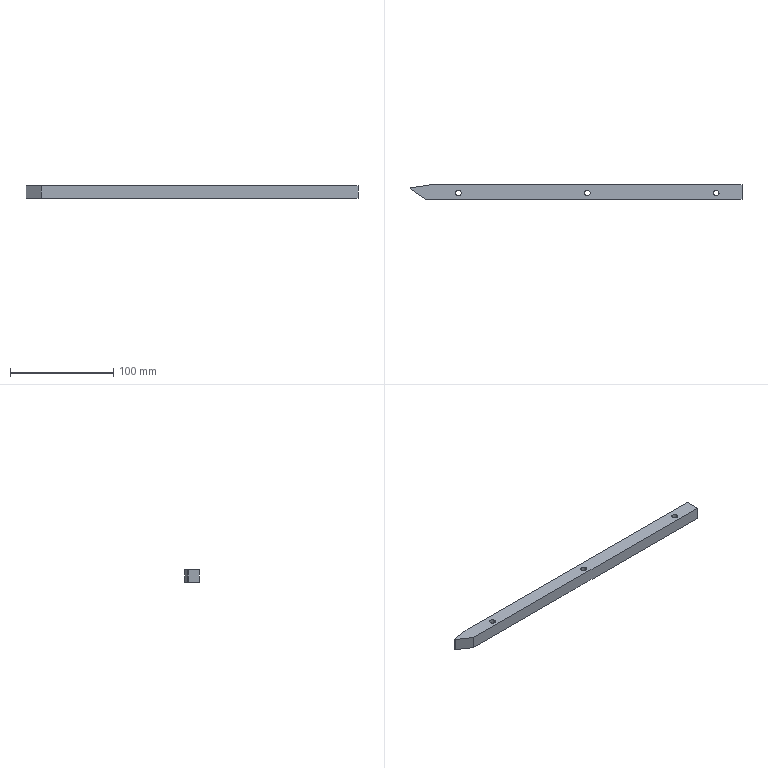Component | SolidWorks | OPW-05-014-1 | 1 solid | 23 faces | box 322 x 14 x 12 mm | volume 51159 mm3 | cylinder 12 | plane 11 | commonest cylinder face diameters 10 x6 5.5 x6
build123d program:
from build123d import *

# Parameters (mm, degrees)
SKETCH1_W                                       = 322
SKETCH1_H                                       = 14
BOSS_EXTRUDE1_DEPTH                             = 6
M5_HEX_SOCKET_HEAD_CAP_SCREW_CBORE1_D           = 5.5
M5_HEX_SOCKET_HEAD_CAP_SCREW_CBORE1_CBORE_D     = 10
M5_HEX_SOCKET_HEAD_CAP_SCREW_CBORE1_CBORE_DEPTH = 5
CHAMFER1_SIZE                                   = 3
CHAMFER1_SIZE2                                  = 20
CUT_EXTRUDE2_REACH                              = 163.598


with BuildPart() as part:
    # Sketch1 → Boss-Extrude1 (new, symmetric)
    with BuildSketch(Plane.XY):
        Rectangle(SKETCH1_W, SKETCH1_H)
    extrude(amount=BOSS_EXTRUDE1_DEPTH, both=True)

    # M5 Hex Socket Head Cap Screw CBORE1 (through all)
    with Locations(Plane.XY.offset(6)):
        with Locations((-136, -1), (-11, -1), (114, -1)):
            CounterBoreHole(M5_HEX_SOCKET_HEAD_CAP_SCREW_CBORE1_D / 2, M5_HEX_SOCKET_HEAD_CAP_SCREW_CBORE1_CBORE_D / 2, M5_HEX_SOCKET_HEAD_CAP_SCREW_CBORE1_CBORE_DEPTH)

    # Chamfer1
    chamfer1_edges = [part.edges().sort_by_distance(p)[0] for p in [
        (161, 7, 0),
    ]]
    chamfer1_side = [part.faces().sort_by_distance(p)[0] for p in [
        (161, 0, 0),
    ]]
    chamfer(chamfer1_edges, length=CHAMFER1_SIZE, length2=CHAMFER1_SIZE2, reference=chamfer1_side[0])

    # Sketch5 → Cut-Extrude2 (cut, up to next)
    with BuildSketch(Plane.XY.offset(6), mode=Mode.PRIVATE) as cut_extrude2_sk1:
        Polygon((161, 3), (146, -7), (161, -7), align=None)
    cut_extrude2_tool1 = extrude(cut_extrude2_sk1.sketch, amount=-CUT_EXTRUDE2_REACH, mode=Mode.PRIVATE) & part.part
    add(cut_extrude2_tool1.solids().sort_by_distance((156, -3.667, 6))[0], mode=Mode.SUBTRACT)


solid = part.part

# Placed as in the assembly
solid = solid.moved(Location((-115.904, 61.999, -46), (-180, 0, 180)))
STEP:
#1=CARTESIAN_POINT('',(0.988,2.402,-1.85));
#2=VERTEX_POINT('',#1);
#3=CARTESIAN_POINT('',(0.5943,2.402,-1.85));
#4=VERTEX_POINT('',#3);
#5=CARTESIAN_POINT('',(0.7912,2.402,-1.85));
#6=DIRECTION('',(-0.,-0.,-1.));
#7=DIRECTION('',(-1.,0.,0.));
#8=AXIS2_PLACEMENT_3D('',#5,#6,#7);
#9=CIRCLE('',#8,0.1969);
#10=EDGE_CURVE('',#2,#4,#9,.T.);
#11=ORIENTED_EDGE('',*,*,#10,.F.);
#12=CARTESIAN_POINT('',(0.988,2.402,-2.047));
#13=VERTEX_POINT('',#12);
#14=CARTESIAN_POINT('',(0.988,2.402,-2.047));
#15=DIRECTION('',(-0.,-0.,-1.));
#16=VECTOR('',#15,39.37);
#17=LINE('',#14,#16);
#18=EDGE_CURVE('',#2,#13,#17,.T.);
#19=ORIENTED_EDGE('',*,*,#18,.T.);
#20=CARTESIAN_POINT('',(0.5943,2.402,-2.047));
#21=VERTEX_POINT('',#20);
#22=CARTESIAN_POINT('',(0.7912,2.402,-2.047));
#23=DIRECTION('',(-0.,-0.,-1.));
#24=DIRECTION('',(-1.,0.,0.));
#25=AXIS2_PLACEMENT_3D('',#22,#23,#24);
#26=CIRCLE('',#25,0.1969);
#27=EDGE_CURVE('',#13,#21,#26,.T.);
#28=ORIENTED_EDGE('',*,*,#27,.T.);
#29=CARTESIAN_POINT('',(0.5943,2.402,-2.047));
#30=DIRECTION('',(-0.,-0.,-1.));
#31=VECTOR('',#30,39.37);
#32=LINE('',#29,#31);
#33=EDGE_CURVE('',#4,#21,#32,.T.);
#34=ORIENTED_EDGE('',*,*,#33,.F.);
#35=EDGE_LOOP('',(#11,#19,#28,#34));
#36=FACE_OUTER_BOUND('',#35,.T.);
#37=CARTESIAN_POINT('',(0.7912,2.402,-2.047));
#38=DIRECTION('',(-0.,-0.,-1.));
#39=DIRECTION('',(-1.,0.,0.));
#40=AXIS2_PLACEMENT_3D('',#37,#38,#39);
#41=CYLINDRICAL_SURFACE('',#40,0.1969);
#42=ADVANCED_FACE('',(#36),#41,.F.);
#43=CARTESIAN_POINT('',(0.8995,2.402,-1.575));
#44=VERTEX_POINT('',#43);
#45=CARTESIAN_POINT('',(0.6829,2.402,-1.575));
#46=VERTEX_POINT('',#45);
#47=CARTESIAN_POINT('',(0.7912,2.402,-1.575));
#48=DIRECTION('',(-0.,-0.,-1.));
#49=DIRECTION('',(-1.,0.,0.));
#50=AXIS2_PLACEMENT_3D('',#47,#48,#49);
#51=CIRCLE('',#50,0.1083);
#52=EDGE_CURVE('',#44,#46,#51,.T.);
#53=ORIENTED_EDGE('',*,*,#52,.F.);
#54=CARTESIAN_POINT('',(0.8995,2.402,-1.85));
#55=VERTEX_POINT('',#54);
#56=CARTESIAN_POINT('',(0.8995,2.402,-2.047));
#57=DIRECTION('',(-0.,-0.,-1.));
#58=VECTOR('',#57,39.37);
#59=LINE('',#56,#58);
#60=EDGE_CURVE('',#44,#55,#59,.T.);
#61=ORIENTED_EDGE('',*,*,#60,.T.);
#62=CARTESIAN_POINT('',(0.6829,2.402,-1.85));
#63=VERTEX_POINT('',#62);
#64=CARTESIAN_POINT('',(0.7912,2.402,-1.85));
#65=DIRECTION('',(-0.,-0.,-1.));
#66=DIRECTION('',(-1.,0.,0.));
#67=AXIS2_PLACEMENT_3D('',#64,#65,#66);
#68=CIRCLE('',#67,0.1083);
#69=EDGE_CURVE('',#55,#63,#68,.T.);
#70=ORIENTED_EDGE('',*,*,#69,.T.);
#71=CARTESIAN_POINT('',(0.6829,2.402,-2.047));
#72=DIRECTION('',(-0.,-0.,-1.));
#73=VECTOR('',#72,39.37);
#74=LINE('',#71,#73);
#75=EDGE_CURVE('',#46,#63,#74,.T.);
#76=ORIENTED_EDGE('',*,*,#75,.F.);
#77=EDGE_LOOP('',(#53,#61,#70,#76));
#78=FACE_OUTER_BOUND('',#77,.T.);
#79=CARTESIAN_POINT('',(0.7912,2.402,-2.047));
#80=DIRECTION('',(-0.,-0.,-1.));
#81=DIRECTION('',(-1.,0.,0.));
#82=AXIS2_PLACEMENT_3D('',#79,#80,#81);
#83=CYLINDRICAL_SURFACE('',#82,0.1083);
#84=ADVANCED_FACE('',(#78),#83,.F.);
#85=CARTESIAN_POINT('',(-3.933,2.402,-1.85));
#86=VERTEX_POINT('',#85);
#87=CARTESIAN_POINT('',(-4.327,2.402,-1.85));
#88=VERTEX_POINT('',#87);
#89=CARTESIAN_POINT('',(-4.13,2.402,-1.85));
#90=DIRECTION('',(-0.,-0.,-1.));
#91=DIRECTION('',(-1.,0.,0.));
#92=AXIS2_PLACEMENT_3D('',#89,#90,#91);
#93=CIRCLE('',#92,0.1969);
#94=EDGE_CURVE('',#86,#88,#93,.T.);
#95=ORIENTED_EDGE('',*,*,#94,.F.);
#96=CARTESIAN_POINT('',(-3.933,2.402,-2.047));
#97=VERTEX_POINT('',#96);
#98=CARTESIAN_POINT('',(-3.933,2.402,-2.047));
#99=DIRECTION('',(-0.,-0.,-1.));
#100=VECTOR('',#99,39.37);
#101=LINE('',#98,#100);
#102=EDGE_CURVE('',#86,#97,#101,.T.);
#103=ORIENTED_EDGE('',*,*,#102,.T.);
#104=CARTESIAN_POINT('',(-4.327,2.402,-2.047));
#105=VERTEX_POINT('',#104);
#106=CARTESIAN_POINT('',(-4.13,2.402,-2.047));
#107=DIRECTION('',(-0.,-0.,-1.));
#108=DIRECTION('',(-1.,0.,0.));
#109=AXIS2_PLACEMENT_3D('',#106,#107,#108);
#110=CIRCLE('',#109,0.1969);
#111=EDGE_CURVE('',#97,#105,#110,.T.);
#112=ORIENTED_EDGE('',*,*,#111,.T.);
#113=CARTESIAN_POINT('',(-4.327,2.402,-2.047));
#114=DIRECTION('',(-0.,-0.,-1.));
#115=VECTOR('',#114,39.37);
#116=LINE('',#113,#115);
#117=EDGE_CURVE('',#88,#105,#116,.T.);
#118=ORIENTED_EDGE('',*,*,#117,.F.);
#119=EDGE_LOOP('',(#95,#103,#112,#118));
#120=FACE_OUTER_BOUND('',#119,.T.);
#121=CARTESIAN_POINT('',(-4.13,2.402,-2.047));
#122=DIRECTION('',(-0.,-0.,-1.));
#123=DIRECTION('',(-1.,0.,0.));
#124=AXIS2_PLACEMENT_3D('',#121,#122,#123);
#125=CYLINDRICAL_SURFACE('',#124,0.1969);
#126=ADVANCED_FACE('',(#120),#125,.F.);
#127=CARTESIAN_POINT('',(-4.022,2.402,-1.575));
#128=VERTEX_POINT('',#127);
#129=CARTESIAN_POINT('',(-4.238,2.402,-1.575));
#130=VERTEX_POINT('',#129);
#131=CARTESIAN_POINT('',(-4.13,2.402,-1.575));
#132=DIRECTION('',(-0.,-0.,-1.));
#133=DIRECTION('',(-1.,0.,0.));
#134=AXIS2_PLACEMENT_3D('',#131,#132,#133);
#135=CIRCLE('',#134,0.1083);
#136=EDGE_CURVE('',#128,#130,#135,.T.);
#137=ORIENTED_EDGE('',*,*,#136,.F.);
#138=CARTESIAN_POINT('',(-4.022,2.402,-1.85));
#139=VERTEX_POINT('',#138);
#140=CARTESIAN_POINT('',(-4.022,2.402,-2.047));
#141=DIRECTION('',(-0.,-0.,-1.));
#142=VECTOR('',#141,39.37);
#143=LINE('',#140,#142);
#144=EDGE_CURVE('',#128,#139,#143,.T.);
#145=ORIENTED_EDGE('',*,*,#144,.T.);
#146=CARTESIAN_POINT('',(-4.238,2.402,-1.85));
#147=VERTEX_POINT('',#146);
#148=CARTESIAN_POINT('',(-4.13,2.402,-1.85));
#149=DIRECTION('',(-0.,-0.,-1.));
#150=DIRECTION('',(-1.,0.,0.));
#151=AXIS2_PLACEMENT_3D('',#148,#149,#150);
#152=CIRCLE('',#151,0.1083);
#153=EDGE_CURVE('',#139,#147,#152,.T.);
#154=ORIENTED_EDGE('',*,*,#153,.T.);
#155=CARTESIAN_POINT('',(-4.238,2.402,-2.047));
#156=DIRECTION('',(-0.,-0.,-1.));
#157=VECTOR('',#156,39.37);
#158=LINE('',#155,#157);
#159=EDGE_CURVE('',#130,#147,#158,.T.);
#160=ORIENTED_EDGE('',*,*,#159,.F.);
#161=EDGE_LOOP('',(#137,#145,#154,#160));
#162=FACE_OUTER_BOUND('',#161,.T.);
#163=CARTESIAN_POINT('',(-4.13,2.402,-2.047));
#164=DIRECTION('',(-0.,-0.,-1.));
#165=DIRECTION('',(-1.,0.,0.));
#166=AXIS2_PLACEMENT_3D('',#163,#164,#165);
#167=CYLINDRICAL_SURFACE('',#166,0.1083);
#168=ADVANCED_FACE('',(#162),#167,.F.);
#169=CARTESIAN_POINT('',(-8.854,2.402,-1.85));
#170=VERTEX_POINT('',#169);
#171=CARTESIAN_POINT('',(-9.248,2.402,-1.85));
#172=VERTEX_POINT('',#171);
#173=CARTESIAN_POINT('',(-9.051,2.402,-1.85));
#174=DIRECTION('',(-0.,-0.,-1.));
#175=DIRECTION('',(-1.,0.,0.));
#176=AXIS2_PLACEMENT_3D('',#173,#174,#175);
#177=CIRCLE('',#176,0.1969);
#178=EDGE_CURVE('',#170,#172,#177,.T.);
#179=ORIENTED_EDGE('',*,*,#178,.F.);
#180=CARTESIAN_POINT('',(-8.854,2.402,-2.047));
#181=VERTEX_POINT('',#180);
#182=CARTESIAN_POINT('',(-8.854,2.402,-2.047));
#183=DIRECTION('',(-0.,-0.,-1.));
#184=VECTOR('',#183,39.37);
#185=LINE('',#182,#184);
#186=EDGE_CURVE('',#170,#181,#185,.T.);
#187=ORIENTED_EDGE('',*,*,#186,.T.);
#188=CARTESIAN_POINT('',(-9.248,2.402,-2.047));
#189=VERTEX_POINT('',#188);
#190=CARTESIAN_POINT('',(-9.051,2.402,-2.047));
#191=DIRECTION('',(-0.,-0.,-1.));
#192=DIRECTION('',(-1.,0.,0.));
#193=AXIS2_PLACEMENT_3D('',#190,#191,#192);
#194=CIRCLE('',#193,0.1969);
#195=EDGE_CURVE('',#181,#189,#194,.T.);
#196=ORIENTED_EDGE('',*,*,#195,.T.);
#197=CARTESIAN_POINT('',(-9.248,2.402,-2.047));
#198=DIRECTION('',(-0.,-0.,-1.));
#199=VECTOR('',#198,39.37);
#200=LINE('',#197,#199);
#201=EDGE_CURVE('',#172,#189,#200,.T.);
#202=ORIENTED_EDGE('',*,*,#201,.F.);
#203=EDGE_LOOP('',(#179,#187,#196,#202));
#204=FACE_OUTER_BOUND('',#203,.T.);
#205=CARTESIAN_POINT('',(-9.051,2.402,-2.047));
#206=DIRECTION('',(-0.,-0.,-1.));
#207=DIRECTION('',(-1.,0.,0.));
#208=AXIS2_PLACEMENT_3D('',#205,#206,#207);
#209=CYLINDRICAL_SURFACE('',#208,0.1969);
#210=ADVANCED_FACE('',(#204),#209,.F.);
#211=CARTESIAN_POINT('',(-8.943,2.402,-1.575));
#212=VERTEX_POINT('',#211);
#213=CARTESIAN_POINT('',(-9.16,2.402,-1.575));
#214=VERTEX_POINT('',#213);
#215=CARTESIAN_POINT('',(-9.051,2.402,-1.575));
#216=DIRECTION('',(-0.,-0.,-1.));
#217=DIRECTION('',(-1.,0.,0.));
#218=AXIS2_PLACEMENT_3D('',#215,#216,#217);
#219=CIRCLE('',#218,0.1083);
#220=EDGE_CURVE('',#212,#214,#219,.T.);
#221=ORIENTED_EDGE('',*,*,#220,.F.);
#222=CARTESIAN_POINT('',(-8.943,2.402,-1.85));
#223=VERTEX_POINT('',#222);
#224=CARTESIAN_POINT('',(-8.943,2.402,-2.047));
#225=DIRECTION('',(-0.,-0.,-1.));
#226=VECTOR('',#225,39.37);
#227=LINE('',#224,#226);
#228=EDGE_CURVE('',#212,#223,#227,.T.);
#229=ORIENTED_EDGE('',*,*,#228,.T.);
#230=CARTESIAN_POINT('',(-9.16,2.402,-1.85));
#231=VERTEX_POINT('',#230);
#232=CARTESIAN_POINT('',(-9.051,2.402,-1.85));
#233=DIRECTION('',(-0.,-0.,-1.));
#234=DIRECTION('',(-1.,0.,0.));
#235=AXIS2_PLACEMENT_3D('',#232,#233,#234);
#236=CIRCLE('',#235,0.1083);
#237=EDGE_CURVE('',#223,#231,#236,.T.);
#238=ORIENTED_EDGE('',*,*,#237,.T.);
#239=CARTESIAN_POINT('',(-9.16,2.402,-2.047));
#240=DIRECTION('',(-0.,-0.,-1.));
#241=VECTOR('',#240,39.37);
#242=LINE('',#239,#241);
#243=EDGE_CURVE('',#214,#231,#242,.T.);
#244=ORIENTED_EDGE('',*,*,#243,.F.);
#245=EDGE_LOOP('',(#221,#229,#238,#244));
#246=FACE_OUTER_BOUND('',#245,.T.);
#247=CARTESIAN_POINT('',(-9.051,2.402,-2.047));
#248=DIRECTION('',(-0.,-0.,-1.));
#249=DIRECTION('',(-1.,0.,0.));
#250=AXIS2_PLACEMENT_3D('',#247,#248,#249);
#251=CYLINDRICAL_SURFACE('',#250,0.1083);
#252=ADVANCED_FACE('',(#246),#251,.F.);
#253=CARTESIAN_POINT('',(1.775,2.716,-1.575));
#254=VERTEX_POINT('',#253);
#255=CARTESIAN_POINT('',(1.775,2.165,-1.575));
#256=VERTEX_POINT('',#255);
#257=CARTESIAN_POINT('',(1.775,2.716,-1.575));
#258=DIRECTION('',(-0.,-1.,0.));
#259=VECTOR('',#258,39.37);
#260=LINE('',#257,#259);
#261=EDGE_CURVE('',#254,#256,#260,.T.);
#262=ORIENTED_EDGE('',*,*,#261,.T.);
#263=CARTESIAN_POINT('',(1.775,2.165,-2.047));
#264=VERTEX_POINT('',#263);
#265=CARTESIAN_POINT('',(1.775,2.165,-2.047));
#266=DIRECTION('',(0.,0.,1.));
#267=VECTOR('',#266,39.37);
#268=LINE('',#265,#267);
#269=EDGE_CURVE('',#264,#256,#268,.T.);
#270=ORIENTED_EDGE('',*,*,#269,.F.);
#271=CARTESIAN_POINT('',(1.775,2.716,-2.047));
#272=VERTEX_POINT('',#271);
#273=CARTESIAN_POINT('',(1.775,2.716,-2.047));
#274=DIRECTION('',(-0.,-1.,0.));
#275=VECTOR('',#274,39.37);
#276=LINE('',#273,#275);
#277=EDGE_CURVE('',#272,#264,#276,.T.);
#278=ORIENTED_EDGE('',*,*,#277,.F.);
#279=CARTESIAN_POINT('',(1.775,2.716,-2.047));
#280=DIRECTION('',(0.,0.,1.));
#281=VECTOR('',#280,39.37);
#282=LINE('',#279,#281);
#283=EDGE_CURVE('',#272,#254,#282,.T.);
#284=ORIENTED_EDGE('',*,*,#283,.T.);
#285=EDGE_LOOP('',(#262,#270,#278,#284));
#286=FACE_OUTER_BOUND('',#285,.T.);
#287=CARTESIAN_POINT('',(1.775,2.716,-2.047));
#288=DIRECTION('',(-1.,0.,0.));
#289=DIRECTION('',(0.,0.,1.));
#290=AXIS2_PLACEMENT_3D('',#287,#288,#289);
#291=PLANE('',#290);
#292=ADVANCED_FACE('',(#286),#291,.F.);
#293=CARTESIAN_POINT('',(-10.311,2.165,-1.575));
#294=VERTEX_POINT('',#293);
#295=CARTESIAN_POINT('',(1.775,2.165,-1.575));
#296=DIRECTION('',(-1.,0.,-0.));
#297=VECTOR('',#296,39.37);
#298=LINE('',#295,#297);
#299=EDGE_CURVE('',#256,#294,#298,.T.);
#300=ORIENTED_EDGE('',*,*,#299,.T.);
#301=CARTESIAN_POINT('',(-10.311,2.165,-2.047));
#302=VERTEX_POINT('',#301);
#303=CARTESIAN_POINT('',(-10.311,2.165,-1.575));
#304=DIRECTION('',(-0.,-0.,-1.));
#305=VECTOR('',#304,39.37);
#306=LINE('',#303,#305);
#307=EDGE_CURVE('',#294,#302,#306,.T.);
#308=ORIENTED_EDGE('',*,*,#307,.T.);
#309=CARTESIAN_POINT('',(1.775,2.165,-2.047));
#310=DIRECTION('',(-1.,0.,-0.));
#311=VECTOR('',#310,39.37);
#312=LINE('',#309,#311);
#313=EDGE_CURVE('',#264,#302,#312,.T.);
#314=ORIENTED_EDGE('',*,*,#313,.F.);
#315=ORIENTED_EDGE('',*,*,#269,.T.);
#316=EDGE_LOOP('',(#300,#308,#314,#315));
#317=FACE_OUTER_BOUND('',#316,.T.);
#318=CARTESIAN_POINT('',(1.775,2.165,-2.047));
#319=DIRECTION('',(0.,1.,-0.));
#320=DIRECTION('',(1.,-0.,0.));
#321=AXIS2_PLACEMENT_3D('',#318,#319,#320);
#322=PLANE('',#321);
#323=ADVANCED_FACE('',(#317),#322,.F.);
#324=CARTESIAN_POINT('',(-10.902,2.559,-2.047));
#325=VERTEX_POINT('',#324);
#326=CARTESIAN_POINT('',(-10.902,2.598,-2.047));
#327=VERTEX_POINT('',#326);
#328=CARTESIAN_POINT('',(-10.902,2.716,-2.047));
#329=DIRECTION('',(0.,1.,-0.));
#330=VECTOR('',#329,39.37);
#331=LINE('',#328,#330);
#332=EDGE_CURVE('',#325,#327,#331,.T.);
#333=ORIENTED_EDGE('',*,*,#332,.F.);
#334=CARTESIAN_POINT('',(-10.902,2.559,-1.575));
#335=VERTEX_POINT('',#334);
#336=CARTESIAN_POINT('',(-10.902,2.559,-1.575));
#337=DIRECTION('',(-0.,-0.,-1.));
#338=VECTOR('',#337,39.37);
#339=LINE('',#336,#338);
#340=EDGE_CURVE('',#335,#325,#339,.T.);
#341=ORIENTED_EDGE('',*,*,#340,.F.);
#342=CARTESIAN_POINT('',(-10.902,2.598,-1.575));
#343=VERTEX_POINT('',#342);
#344=CARTESIAN_POINT('',(-10.902,2.716,-1.575));
#345=DIRECTION('',(0.,1.,-0.));
#346=VECTOR('',#345,39.37);
#347=LINE('',#344,#346);
#348=EDGE_CURVE('',#335,#343,#347,.T.);
#349=ORIENTED_EDGE('',*,*,#348,.T.);
#350=CARTESIAN_POINT('',(-10.902,2.598,-2.047));
#351=DIRECTION('',(-0.,-0.,-1.));
#352=VECTOR('',#351,39.37);
#353=LINE('',#350,#352);
#354=EDGE_CURVE('',#343,#327,#353,.T.);
#355=ORIENTED_EDGE('',*,*,#354,.T.);
#356=EDGE_LOOP('',(#333,#341,#349,#355));
#357=FACE_OUTER_BOUND('',#356,.T.);
#358=CARTESIAN_POINT('',(-10.902,2.716,-2.047));
#359=DIRECTION('',(1.,-0.,-0.));
#360=DIRECTION('',(-0.,-0.,-1.));
#361=AXIS2_PLACEMENT_3D('',#358,#359,#360);
#362=PLANE('',#361);
#363=ADVANCED_FACE('',(#357),#362,.F.);
#364=CARTESIAN_POINT('',(-10.114,2.716,-2.047));
#365=VERTEX_POINT('',#364);
#366=CARTESIAN_POINT('',(1.775,2.716,-2.047));
#367=DIRECTION('',(1.,-0.,0.));
#368=VECTOR('',#367,39.37);
#369=LINE('',#366,#368);
#370=EDGE_CURVE('',#365,#272,#369,.T.);
#371=ORIENTED_EDGE('',*,*,#370,.F.);
#372=CARTESIAN_POINT('',(-10.114,2.716,-1.575));
#373=VERTEX_POINT('',#372);
#374=CARTESIAN_POINT('',(-10.114,2.716,-2.047));
#375=DIRECTION('',(0.,0.,1.));
#376=VECTOR('',#375,39.37);
#377=LINE('',#374,#376);
#378=EDGE_CURVE('',#365,#373,#377,.T.);
#379=ORIENTED_EDGE('',*,*,#378,.T.);
#380=CARTESIAN_POINT('',(1.775,2.716,-1.575));
#381=DIRECTION('',(1.,-0.,0.));
#382=VECTOR('',#381,39.37);
#383=LINE('',#380,#382);
#384=EDGE_CURVE('',#373,#254,#383,.T.);
#385=ORIENTED_EDGE('',*,*,#384,.T.);
#386=ORIENTED_EDGE('',*,*,#283,.F.);
#387=EDGE_LOOP('',(#371,#379,#385,#386));
#388=FACE_OUTER_BOUND('',#387,.T.);
#389=CARTESIAN_POINT('',(1.775,2.716,-2.047));
#390=DIRECTION('',(-0.,-1.,0.));
#391=DIRECTION('',(-1.,0.,-0.));
#392=AXIS2_PLACEMENT_3D('',#389,#390,#391);
#393=PLANE('',#392);
#394=ADVANCED_FACE('',(#388),#393,.F.);
#395=CARTESIAN_POINT('',(-10.902,2.559,-2.047));
#396=DIRECTION('',(0.8321,-0.5547,0.));
#397=VECTOR('',#396,39.37);
#398=LINE('',#395,#397);
#399=EDGE_CURVE('',#325,#302,#398,.T.);
#400=ORIENTED_EDGE('',*,*,#399,.F.);
#401=ORIENTED_EDGE('',*,*,#332,.T.);
#402=CARTESIAN_POINT('',(1.433,4.449,-2.047));
#403=DIRECTION('',(0.9889,0.1483,0.));
#404=VECTOR('',#403,39.37);
#405=LINE('',#402,#404);
#406=EDGE_CURVE('',#327,#365,#405,.T.);
#407=ORIENTED_EDGE('',*,*,#406,.T.);
#408=ORIENTED_EDGE('',*,*,#370,.T.);
#409=ORIENTED_EDGE('',*,*,#277,.T.);
#410=ORIENTED_EDGE('',*,*,#313,.T.);
#411=EDGE_LOOP('',(#400,#401,#407,#408,#409,#410));
#412=FACE_OUTER_BOUND('',#411,.T.);
#413=CARTESIAN_POINT('',(0.7912,2.402,-2.047));
#414=DIRECTION('',(-0.,-0.,-1.));
#415=DIRECTION('',(-1.,0.,0.));
#416=AXIS2_PLACEMENT_3D('',#413,#414,#415);
#417=CIRCLE('',#416,0.1969);
#418=EDGE_CURVE('',#21,#13,#417,.T.);
#419=ORIENTED_EDGE('',*,*,#418,.F.);
#420=ORIENTED_EDGE('',*,*,#27,.F.);
#421=EDGE_LOOP('',(#419,#420));
#422=FACE_BOUND('',#421,.T.);
#423=CARTESIAN_POINT('',(-4.13,2.402,-2.047));
#424=DIRECTION('',(-0.,-0.,-1.));
#425=DIRECTION('',(-1.,0.,0.));
#426=AXIS2_PLACEMENT_3D('',#423,#424,#425);
#427=CIRCLE('',#426,0.1969);
#428=EDGE_CURVE('',#105,#97,#427,.T.);
#429=ORIENTED_EDGE('',*,*,#428,.F.);
#430=ORIENTED_EDGE('',*,*,#111,.F.);
#431=EDGE_LOOP('',(#429,#430));
#432=FACE_BOUND('',#431,.T.);
#433=CARTESIAN_POINT('',(-9.051,2.402,-2.047));
#434=DIRECTION('',(-0.,-0.,-1.));
#435=DIRECTION('',(-1.,0.,0.));
#436=AXIS2_PLACEMENT_3D('',#433,#434,#435);
#437=CIRCLE('',#436,0.1969);
#438=EDGE_CURVE('',#189,#181,#437,.T.);
#439=ORIENTED_EDGE('',*,*,#438,.F.);
#440=ORIENTED_EDGE('',*,*,#195,.F.);
#441=EDGE_LOOP('',(#439,#440));
#442=FACE_BOUND('',#441,.T.);
#443=CARTESIAN_POINT('',(1.775,2.165,-2.047));
#444=DIRECTION('',(0.,-0.,-1.));
#445=DIRECTION('',(-1.,0.,-0.));
#446=AXIS2_PLACEMENT_3D('',#443,#444,#445);
#447=PLANE('',#446);
#448=ADVANCED_FACE('',(#412,#422,#432,#442),#447,.T.);
#449=CARTESIAN_POINT('',(0.7912,2.402,-1.575));
#450=DIRECTION('',(-0.,-0.,-1.));
#451=DIRECTION('',(-1.,0.,0.));
#452=AXIS2_PLACEMENT_3D('',#449,#450,#451);
#453=CIRCLE('',#452,0.1083);
#454=EDGE_CURVE('',#46,#44,#453,.T.);
#455=ORIENTED_EDGE('',*,*,#454,.T.);
#456=ORIENTED_EDGE('',*,*,#52,.T.);
#457=EDGE_LOOP('',(#455,#456));
#458=FACE_BOUND('',#457,.T.);
#459=CARTESIAN_POINT('',(-4.13,2.402,-1.575));
#460=DIRECTION('',(-0.,-0.,-1.));
#461=DIRECTION('',(-1.,0.,0.));
#462=AXIS2_PLACEMENT_3D('',#459,#460,#461);
#463=CIRCLE('',#462,0.1083);
#464=EDGE_CURVE('',#130,#128,#463,.T.);
#465=ORIENTED_EDGE('',*,*,#464,.T.);
#466=ORIENTED_EDGE('',*,*,#136,.T.);
#467=EDGE_LOOP('',(#465,#466));
#468=FACE_BOUND('',#467,.T.);
#469=CARTESIAN_POINT('',(-9.051,2.402,-1.575));
#470=DIRECTION('',(-0.,-0.,-1.));
#471=DIRECTION('',(-1.,0.,0.));
#472=AXIS2_PLACEMENT_3D('',#469,#470,#471);
#473=CIRCLE('',#472,0.1083);
#474=EDGE_CURVE('',#214,#212,#473,.T.);
#475=ORIENTED_EDGE('',*,*,#474,.T.);
#476=ORIENTED_EDGE('',*,*,#220,.T.);
#477=EDGE_LOOP('',(#475,#476));
#478=FACE_BOUND('',#477,.T.);
#479=ORIENTED_EDGE('',*,*,#348,.F.);
#480=CARTESIAN_POINT('',(-10.902,2.559,-1.575));
#481=DIRECTION('',(-0.8321,0.5547,-0.));
#482=VECTOR('',#481,39.37);
#483=LINE('',#480,#482);
#484=EDGE_CURVE('',#294,#335,#483,.T.);
#485=ORIENTED_EDGE('',*,*,#484,.F.);
#486=ORIENTED_EDGE('',*,*,#299,.F.);
#487=ORIENTED_EDGE('',*,*,#261,.F.);
#488=ORIENTED_EDGE('',*,*,#384,.F.);
#489=CARTESIAN_POINT('',(-10.114,2.716,-1.575));
#490=DIRECTION('',(-0.9889,-0.1483,-0.));
#491=VECTOR('',#490,39.37);
#492=LINE('',#489,#491);
#493=EDGE_CURVE('',#373,#343,#492,.T.);
#494=ORIENTED_EDGE('',*,*,#493,.T.);
#495=EDGE_LOOP('',(#479,#485,#486,#487,#488,#494));
#496=FACE_OUTER_BOUND('',#495,.T.);
#497=CARTESIAN_POINT('',(1.775,2.165,-1.575));
#498=DIRECTION('',(0.,-0.,-1.));
#499=DIRECTION('',(-1.,0.,-0.));
#500=AXIS2_PLACEMENT_3D('',#497,#498,#499);
#501=PLANE('',#500);
#502=ADVANCED_FACE('',(#458,#468,#478,#496),#501,.F.);
#503=ORIENTED_EDGE('',*,*,#228,.F.);
#504=ORIENTED_EDGE('',*,*,#474,.F.);
#505=ORIENTED_EDGE('',*,*,#243,.T.);
#506=CARTESIAN_POINT('',(-9.051,2.402,-1.85));
#507=DIRECTION('',(-0.,-0.,-1.));
#508=DIRECTION('',(-1.,0.,0.));
#509=AXIS2_PLACEMENT_3D('',#506,#507,#508);
#510=CIRCLE('',#509,0.1083);
#511=EDGE_CURVE('',#231,#223,#510,.T.);
#512=ORIENTED_EDGE('',*,*,#511,.T.);
#513=EDGE_LOOP('',(#503,#504,#505,#512));
#514=FACE_OUTER_BOUND('',#513,.T.);
#515=CARTESIAN_POINT('',(-9.051,2.402,-2.047));
#516=DIRECTION('',(-0.,-0.,-1.));
#517=DIRECTION('',(-1.,0.,0.));
#518=AXIS2_PLACEMENT_3D('',#515,#516,#517);
#519=CYLINDRICAL_SURFACE('',#518,0.1083);
#520=ADVANCED_FACE('',(#514),#519,.F.);
#521=ORIENTED_EDGE('',*,*,#511,.F.);
#522=ORIENTED_EDGE('',*,*,#237,.F.);
#523=EDGE_LOOP('',(#521,#522));
#524=FACE_BOUND('',#523,.T.);
#525=CARTESIAN_POINT('',(-9.051,2.402,-1.85));
#526=DIRECTION('',(-0.,-0.,-1.));
#527=DIRECTION('',(-1.,0.,0.));
#528=AXIS2_PLACEMENT_3D('',#525,#526,#527);
#529=CIRCLE('',#528,0.1969);
#530=EDGE_CURVE('',#172,#170,#529,.T.);
#531=ORIENTED_EDGE('',*,*,#530,.T.);
#532=ORIENTED_EDGE('',*,*,#178,.T.);
#533=EDGE_LOOP('',(#531,#532));
#534=FACE_OUTER_BOUND('',#533,.T.);
#535=CARTESIAN_POINT('',(-9.16,2.402,-1.85));
#536=DIRECTION('',(-0.,0.,1.));
#537=DIRECTION('',(1.,-0.,0.));
#538=AXIS2_PLACEMENT_3D('',#535,#536,#537);
#539=PLANE('',#538);
#540=ADVANCED_FACE('',(#524,#534),#539,.F.);
#541=ORIENTED_EDGE('',*,*,#186,.F.);
#542=ORIENTED_EDGE('',*,*,#530,.F.);
#543=ORIENTED_EDGE('',*,*,#201,.T.);
#544=ORIENTED_EDGE('',*,*,#438,.T.);
#545=EDGE_LOOP('',(#541,#542,#543,#544));
#546=FACE_OUTER_BOUND('',#545,.T.);
#547=CARTESIAN_POINT('',(-9.051,2.402,-2.047));
#548=DIRECTION('',(-0.,-0.,-1.));
#549=DIRECTION('',(-1.,0.,0.));
#550=AXIS2_PLACEMENT_3D('',#547,#548,#549);
#551=CYLINDRICAL_SURFACE('',#550,0.1969);
#552=ADVANCED_FACE('',(#546),#551,.F.);
#553=ORIENTED_EDGE('',*,*,#144,.F.);
#554=ORIENTED_EDGE('',*,*,#464,.F.);
#555=ORIENTED_EDGE('',*,*,#159,.T.);
#556=CARTESIAN_POINT('',(-4.13,2.402,-1.85));
#557=DIRECTION('',(-0.,-0.,-1.));
#558=DIRECTION('',(-1.,0.,0.));
#559=AXIS2_PLACEMENT_3D('',#556,#557,#558);
#560=CIRCLE('',#559,0.1083);
#561=EDGE_CURVE('',#147,#139,#560,.T.);
#562=ORIENTED_EDGE('',*,*,#561,.T.);
#563=EDGE_LOOP('',(#553,#554,#555,#562));
#564=FACE_OUTER_BOUND('',#563,.T.);
#565=CARTESIAN_POINT('',(-4.13,2.402,-2.047));
#566=DIRECTION('',(-0.,-0.,-1.));
#567=DIRECTION('',(-1.,0.,0.));
#568=AXIS2_PLACEMENT_3D('',#565,#566,#567);
#569=CYLINDRICAL_SURFACE('',#568,0.1083);
#570=ADVANCED_FACE('',(#564),#569,.F.);
#571=ORIENTED_EDGE('',*,*,#561,.F.);
#572=ORIENTED_EDGE('',*,*,#153,.F.);
#573=EDGE_LOOP('',(#571,#572));
#574=FACE_BOUND('',#573,.T.);
#575=CARTESIAN_POINT('',(-4.13,2.402,-1.85));
#576=DIRECTION('',(-0.,-0.,-1.));
#577=DIRECTION('',(-1.,0.,0.));
#578=AXIS2_PLACEMENT_3D('',#575,#576,#577);
#579=CIRCLE('',#578,0.1969);
#580=EDGE_CURVE('',#88,#86,#579,.T.);
#581=ORIENTED_EDGE('',*,*,#580,.T.);
#582=ORIENTED_EDGE('',*,*,#94,.T.);
#583=EDGE_LOOP('',(#581,#582));
#584=FACE_OUTER_BOUND('',#583,.T.);
#585=CARTESIAN_POINT('',(-4.238,2.402,-1.85));
#586=DIRECTION('',(-0.,0.,1.));
#587=DIRECTION('',(1.,-0.,0.));
#588=AXIS2_PLACEMENT_3D('',#585,#586,#587);
#589=PLANE('',#588);
#590=ADVANCED_FACE('',(#574,#584),#589,.F.);
#591=ORIENTED_EDGE('',*,*,#102,.F.);
#592=ORIENTED_EDGE('',*,*,#580,.F.);
#593=ORIENTED_EDGE('',*,*,#117,.T.);
#594=ORIENTED_EDGE('',*,*,#428,.T.);
#595=EDGE_LOOP('',(#591,#592,#593,#594));
#596=FACE_OUTER_BOUND('',#595,.T.);
#597=CARTESIAN_POINT('',(-4.13,2.402,-2.047));
#598=DIRECTION('',(-0.,-0.,-1.));
#599=DIRECTION('',(-1.,0.,0.));
#600=AXIS2_PLACEMENT_3D('',#597,#598,#599);
#601=CYLINDRICAL_SURFACE('',#600,0.1969);
#602=ADVANCED_FACE('',(#596),#601,.F.);
#603=ORIENTED_EDGE('',*,*,#60,.F.);
#604=ORIENTED_EDGE('',*,*,#454,.F.);
#605=ORIENTED_EDGE('',*,*,#75,.T.);
#606=CARTESIAN_POINT('',(0.7912,2.402,-1.85));
#607=DIRECTION('',(-0.,-0.,-1.));
#608=DIRECTION('',(-1.,0.,0.));
#609=AXIS2_PLACEMENT_3D('',#606,#607,#608);
#610=CIRCLE('',#609,0.1083);
#611=EDGE_CURVE('',#63,#55,#610,.T.);
#612=ORIENTED_EDGE('',*,*,#611,.T.);
#613=EDGE_LOOP('',(#603,#604,#605,#612));
#614=FACE_OUTER_BOUND('',#613,.T.);
#615=CARTESIAN_POINT('',(0.7912,2.402,-2.047));
#616=DIRECTION('',(-0.,-0.,-1.));
#617=DIRECTION('',(-1.,0.,0.));
#618=AXIS2_PLACEMENT_3D('',#615,#616,#617);
#619=CYLINDRICAL_SURFACE('',#618,0.1083);
#620=ADVANCED_FACE('',(#614),#619,.F.);
#621=ORIENTED_EDGE('',*,*,#611,.F.);
#622=ORIENTED_EDGE('',*,*,#69,.F.);
#623=EDGE_LOOP('',(#621,#622));
#624=FACE_BOUND('',#623,.T.);
#625=CARTESIAN_POINT('',(0.7912,2.402,-1.85));
#626=DIRECTION('',(-0.,-0.,-1.));
#627=DIRECTION('',(-1.,0.,0.));
#628=AXIS2_PLACEMENT_3D('',#625,#626,#627);
#629=CIRCLE('',#628,0.1969);
#630=EDGE_CURVE('',#4,#2,#629,.T.);
#631=ORIENTED_EDGE('',*,*,#630,.T.);
#632=ORIENTED_EDGE('',*,*,#10,.T.);
#633=EDGE_LOOP('',(#631,#632));
#634=FACE_OUTER_BOUND('',#633,.T.);
#635=CARTESIAN_POINT('',(0.6829,2.402,-1.85));
#636=DIRECTION('',(-0.,0.,1.));
#637=DIRECTION('',(1.,-0.,0.));
#638=AXIS2_PLACEMENT_3D('',#635,#636,#637);
#639=PLANE('',#638);
#640=ADVANCED_FACE('',(#624,#634),#639,.F.);
#641=ORIENTED_EDGE('',*,*,#18,.F.);
#642=ORIENTED_EDGE('',*,*,#630,.F.);
#643=ORIENTED_EDGE('',*,*,#33,.T.);
#644=ORIENTED_EDGE('',*,*,#418,.T.);
#645=EDGE_LOOP('',(#641,#642,#643,#644));
#646=FACE_OUTER_BOUND('',#645,.T.);
#647=CARTESIAN_POINT('',(0.7912,2.402,-2.047));
#648=DIRECTION('',(-0.,-0.,-1.));
#649=DIRECTION('',(-1.,0.,0.));
#650=AXIS2_PLACEMENT_3D('',#647,#648,#649);
#651=CYLINDRICAL_SURFACE('',#650,0.1969);
#652=ADVANCED_FACE('',(#646),#651,.F.);
#653=ORIENTED_EDGE('',*,*,#406,.F.);
#654=ORIENTED_EDGE('',*,*,#354,.F.);
#655=ORIENTED_EDGE('',*,*,#493,.F.);
#656=ORIENTED_EDGE('',*,*,#378,.F.);
#657=EDGE_LOOP('',(#653,#654,#655,#656));
#658=FACE_OUTER_BOUND('',#657,.T.);
#659=CARTESIAN_POINT('',(-10.114,2.716,-2.047));
#660=DIRECTION('',(0.1483,-0.9889,0.));
#661=DIRECTION('',(-0.9889,-0.1483,-0.));
#662=AXIS2_PLACEMENT_3D('',#659,#660,#661);
#663=PLANE('',#662);
#664=ADVANCED_FACE('',(#658),#663,.F.);
#665=ORIENTED_EDGE('',*,*,#484,.T.);
#666=ORIENTED_EDGE('',*,*,#340,.T.);
#667=ORIENTED_EDGE('',*,*,#399,.T.);
#668=ORIENTED_EDGE('',*,*,#307,.F.);
#669=EDGE_LOOP('',(#665,#666,#667,#668));
#670=FACE_OUTER_BOUND('',#669,.T.);
#671=CARTESIAN_POINT('',(-10.902,2.559,-1.575));
#672=DIRECTION('',(0.5547,0.8321,-0.));
#673=DIRECTION('',(0.8321,-0.5547,0.));
#674=AXIS2_PLACEMENT_3D('',#671,#672,#673);
#675=PLANE('',#674);
#676=ADVANCED_FACE('',(#670),#675,.F.);
#677=CLOSED_SHELL('',(#42,#84,#126,#168,#210,#252,#292,#323,#363,#394,#448,#502,#520,#540,#552,#570,#590,#602,#620,#640,#652,#664,#676));
#678=MANIFOLD_SOLID_BREP('',#677);
#679=CARTESIAN_POINT('',(0.,0.,0.));
#680=DIRECTION('',(0.,0.,1.));
#681=DIRECTION('',(1.,0.,0.));
#682=AXIS2_PLACEMENT_3D('',#679,#680,#681);
#683=(LENGTH_UNIT()NAMED_UNIT(*)SI_UNIT($,.METRE.));
#684=LENGTH_MEASURE_WITH_UNIT(LENGTH_MEASURE(0.0254),#683);
#685=DIMENSIONAL_EXPONENTS(1.,0.,0.,0.,0.,0.,0.);
#686=(CONVERSION_BASED_UNIT('',#684)LENGTH_UNIT()NAMED_UNIT(#685));
#687=UNCERTAINTY_MEASURE_WITH_UNIT(LENGTH_MEASURE(0.00001),#686,'','');
#688=(NAMED_UNIT(*)PLANE_ANGLE_UNIT()SI_UNIT($,.RADIAN.));
#689=(NAMED_UNIT(*)SI_UNIT($,.STERADIAN.)SOLID_ANGLE_UNIT());
#690=(GEOMETRIC_REPRESENTATION_CONTEXT(3)GLOBAL_UNCERTAINTY_ASSIGNED_CONTEXT((#687))GLOBAL_UNIT_ASSIGNED_CONTEXT((#686,#688,#689))REPRESENTATION_CONTEXT('',''));
#691=ADVANCED_BREP_SHAPE_REPRESENTATION('',(#678,#682),#690);
#692=COLOUR_RGB('',0.7922,0.8196,0.9333);
#693=FILL_AREA_STYLE_COLOUR('',#692);
#694=FILL_AREA_STYLE('',(#693));
#695=SURFACE_STYLE_FILL_AREA(#694);
#696=SURFACE_SIDE_STYLE('',(#695));
#697=SURFACE_STYLE_USAGE(.BOTH.,#696);
#698=PRESENTATION_STYLE_ASSIGNMENT((#697));
#699=STYLED_ITEM('',(#698),#678);
#700=(LENGTH_UNIT()NAMED_UNIT(*)SI_UNIT($,.METRE.));
#701=LENGTH_MEASURE_WITH_UNIT(LENGTH_MEASURE(0.0254),#700);
#702=DIMENSIONAL_EXPONENTS(1.,0.,0.,0.,0.,0.,0.);
#703=(CONVERSION_BASED_UNIT('',#701)LENGTH_UNIT()NAMED_UNIT(#702));
#704=UNCERTAINTY_MEASURE_WITH_UNIT(LENGTH_MEASURE(0.00001),#703,'','');
#705=(NAMED_UNIT(*)PLANE_ANGLE_UNIT()SI_UNIT($,.RADIAN.));
#706=(NAMED_UNIT(*)SI_UNIT($,.STERADIAN.)SOLID_ANGLE_UNIT());
#707=(GEOMETRIC_REPRESENTATION_CONTEXT(3)GLOBAL_UNCERTAINTY_ASSIGNED_CONTEXT((#704))GLOBAL_UNIT_ASSIGNED_CONTEXT((#703,#705,#706))REPRESENTATION_CONTEXT('',''));
#708=MECHANICAL_DESIGN_GEOMETRIC_PRESENTATION_REPRESENTATION('',(#699),#707);
#709=PRESENTATION_LAYER_ASSIGNMENT('','',(#699));